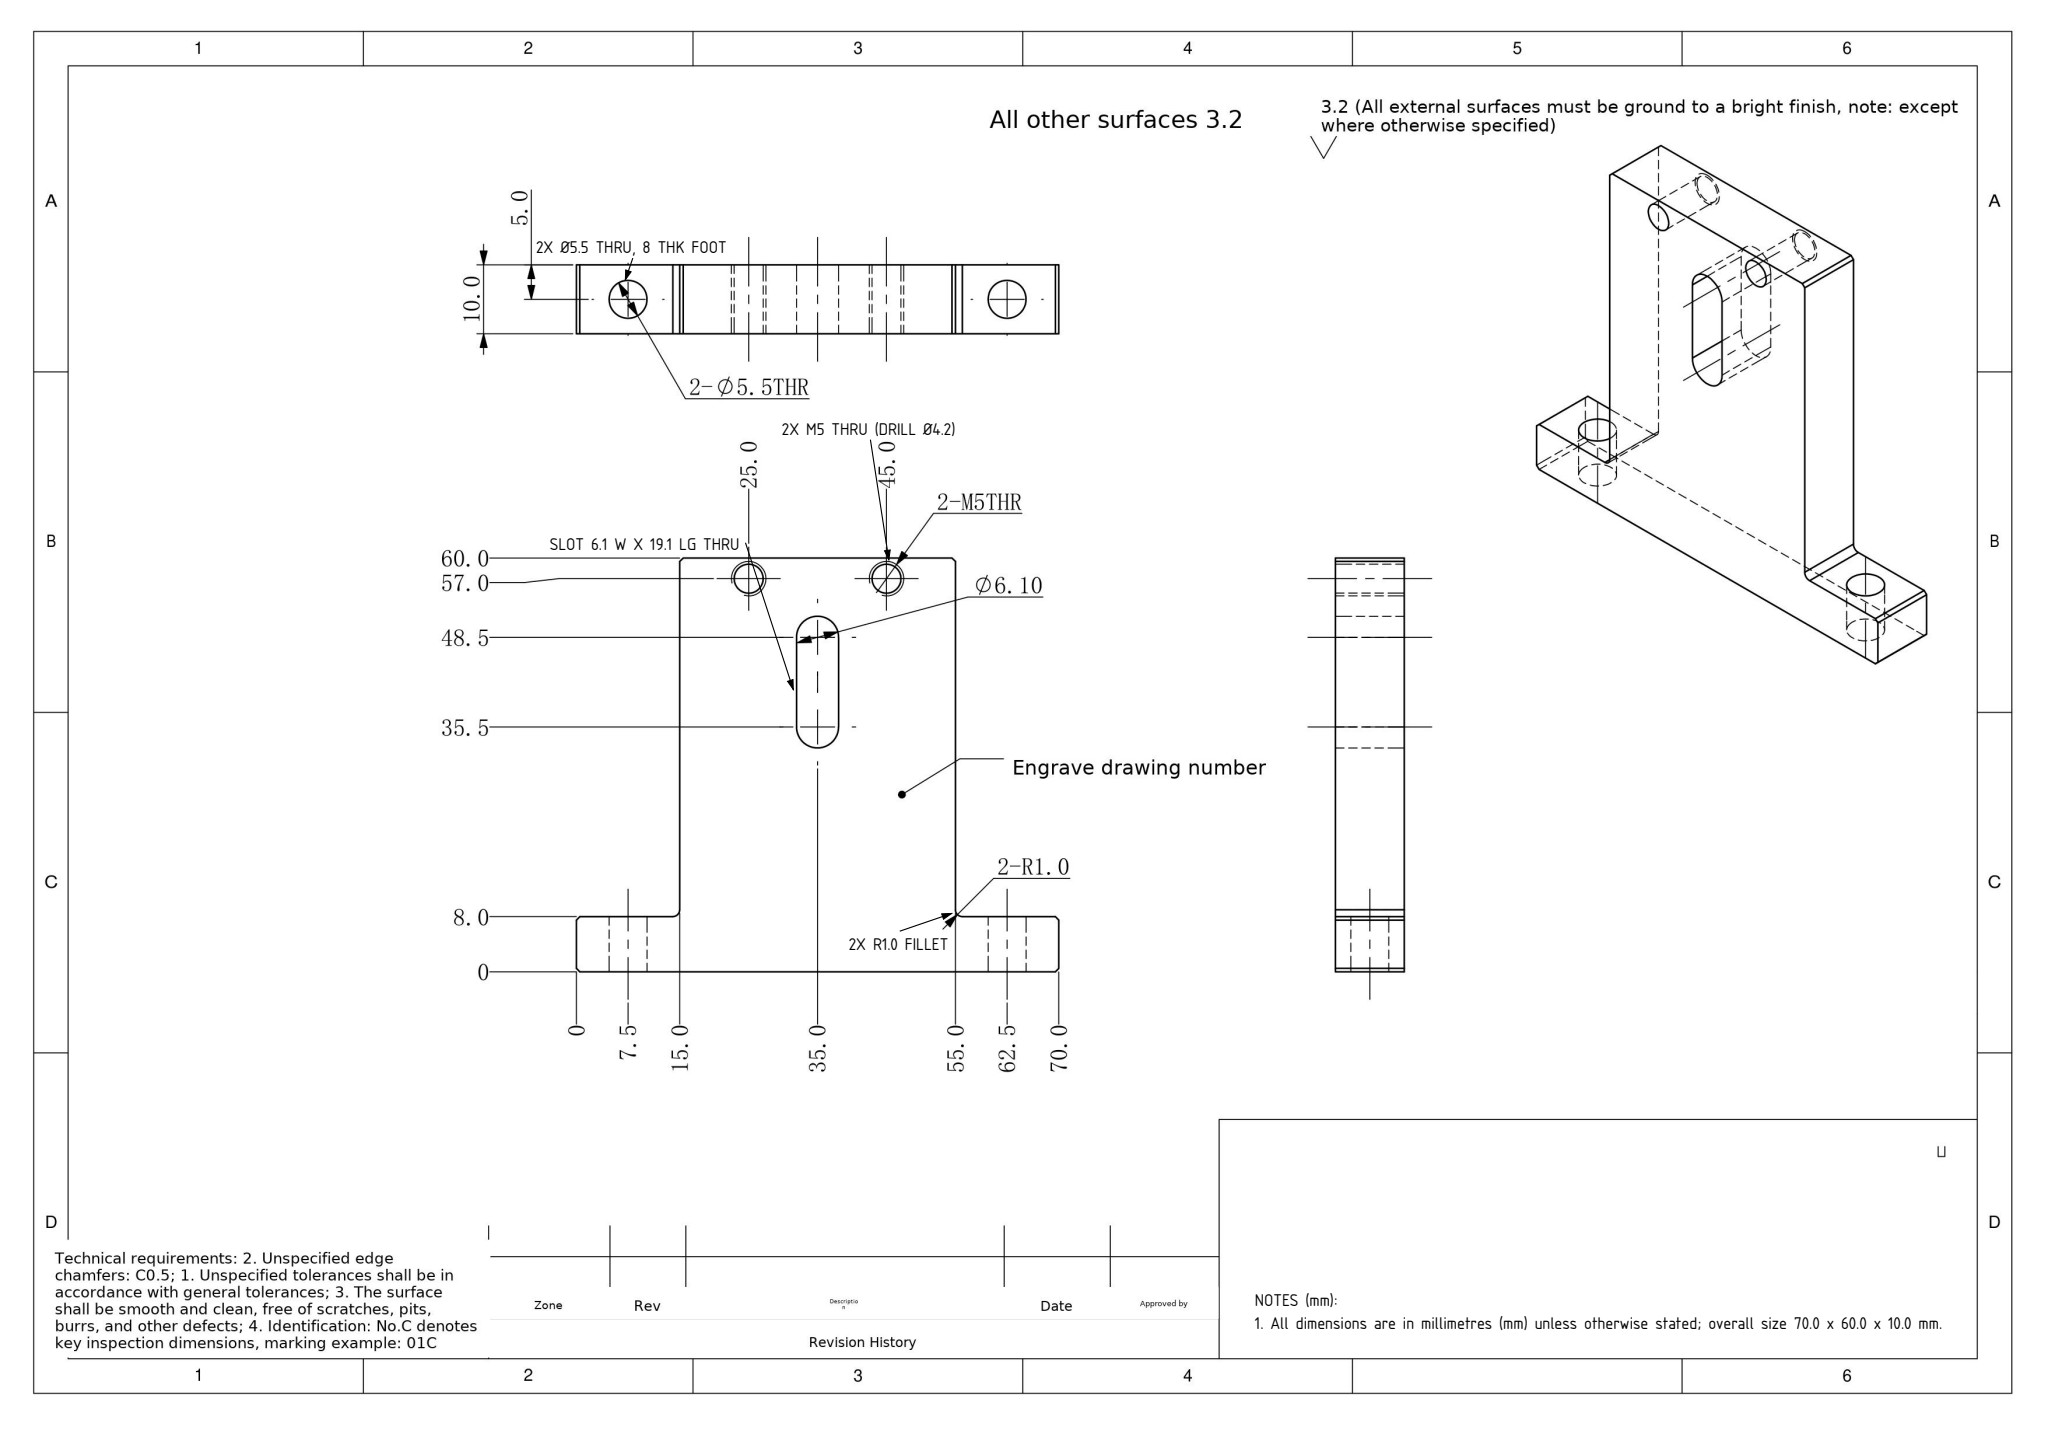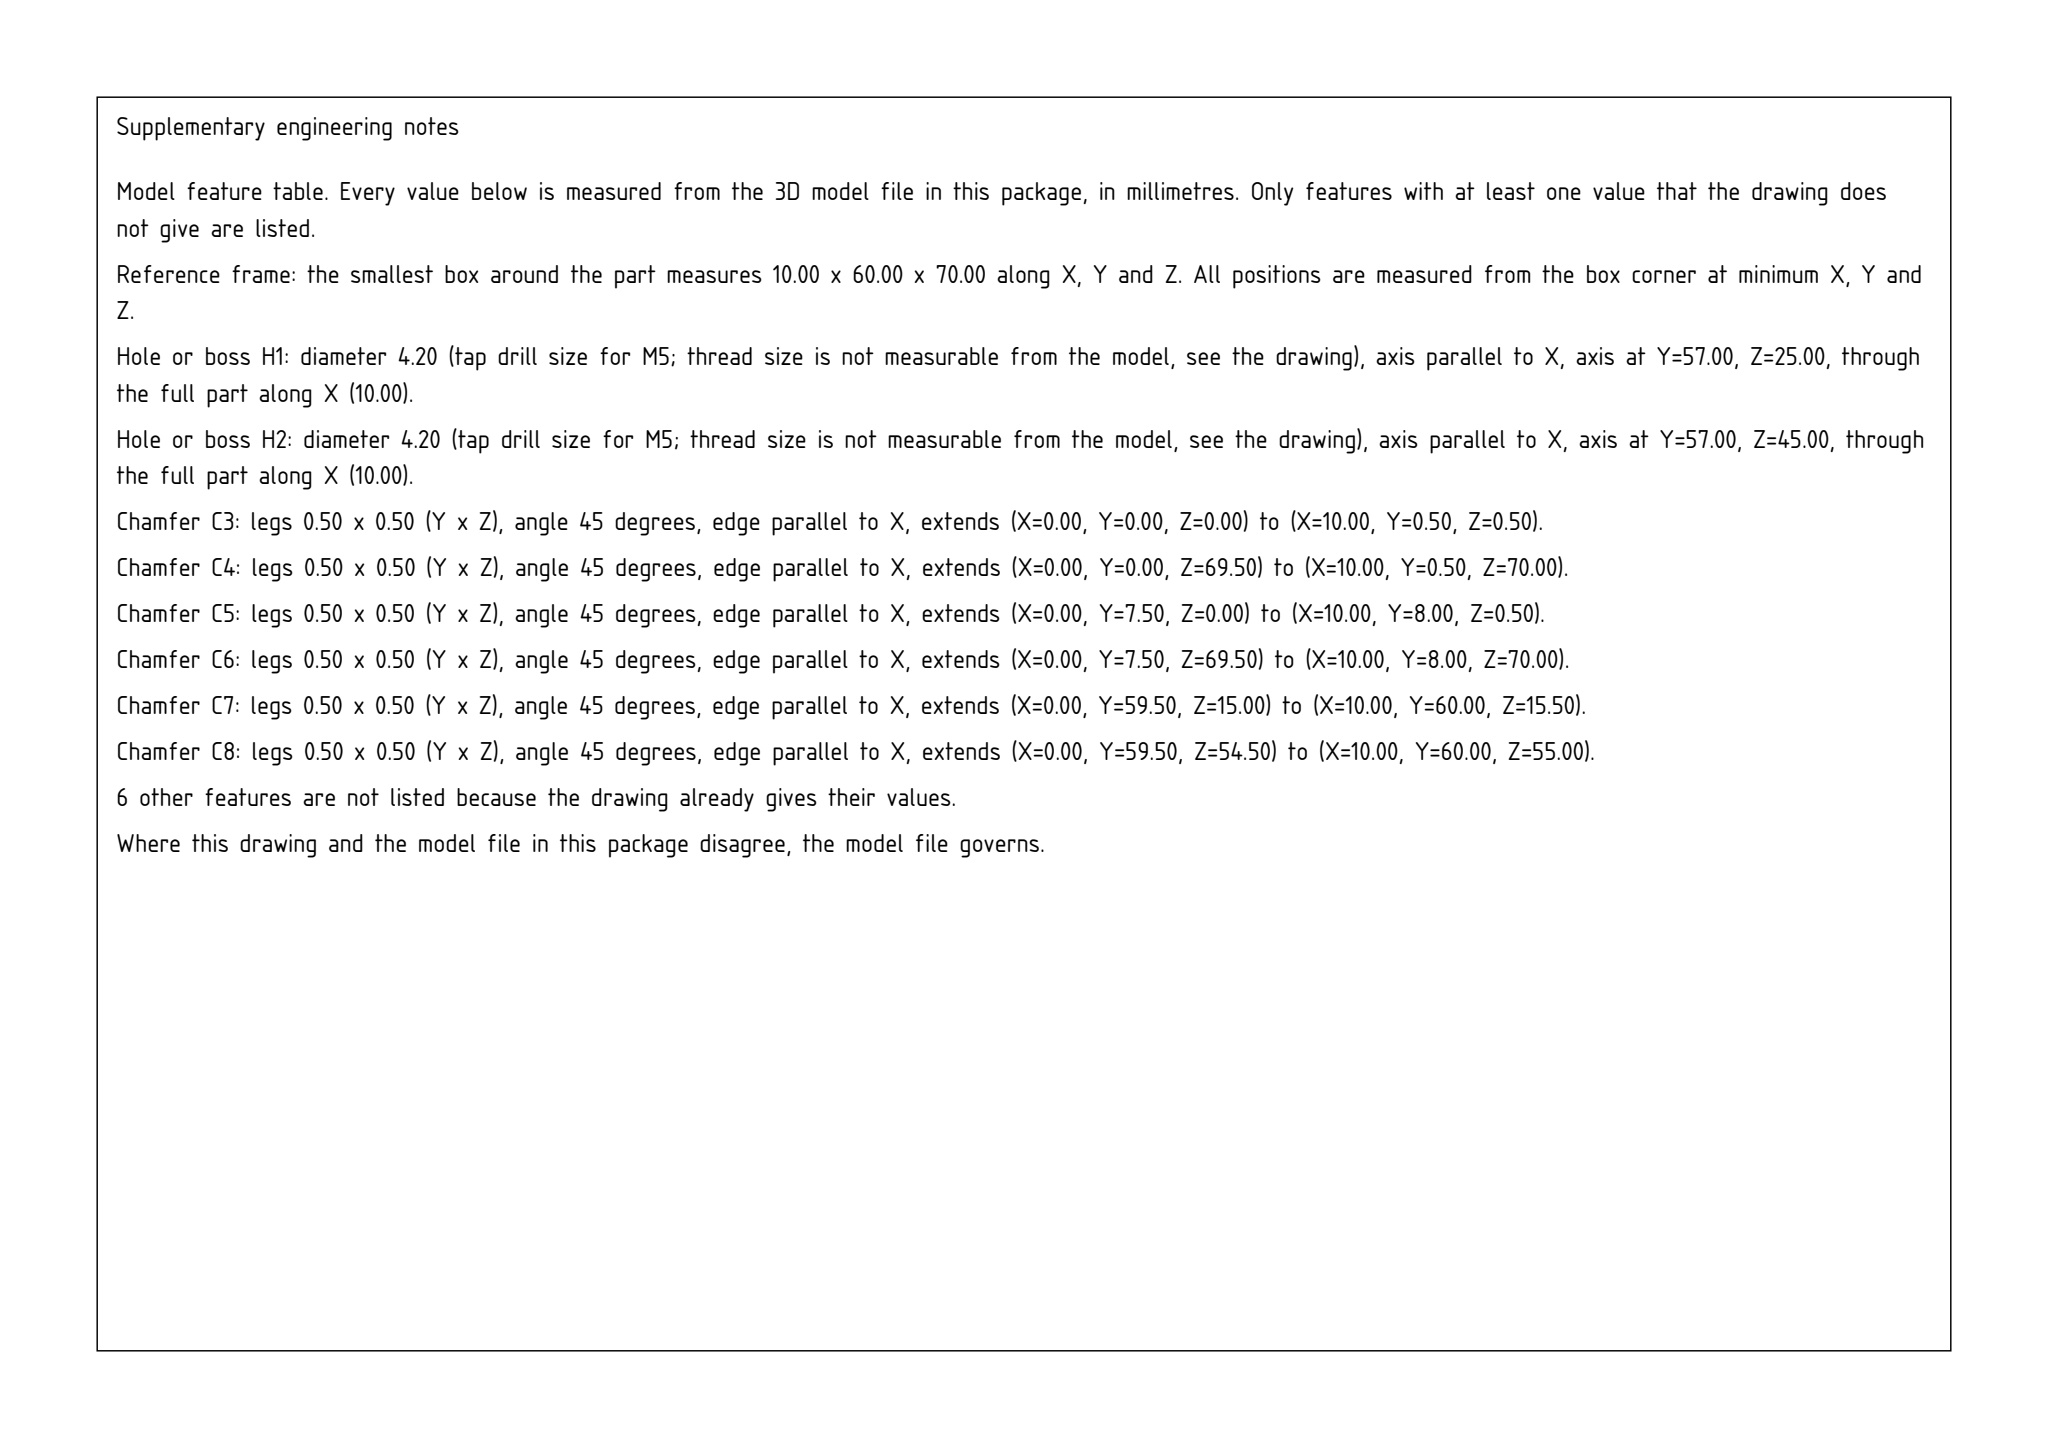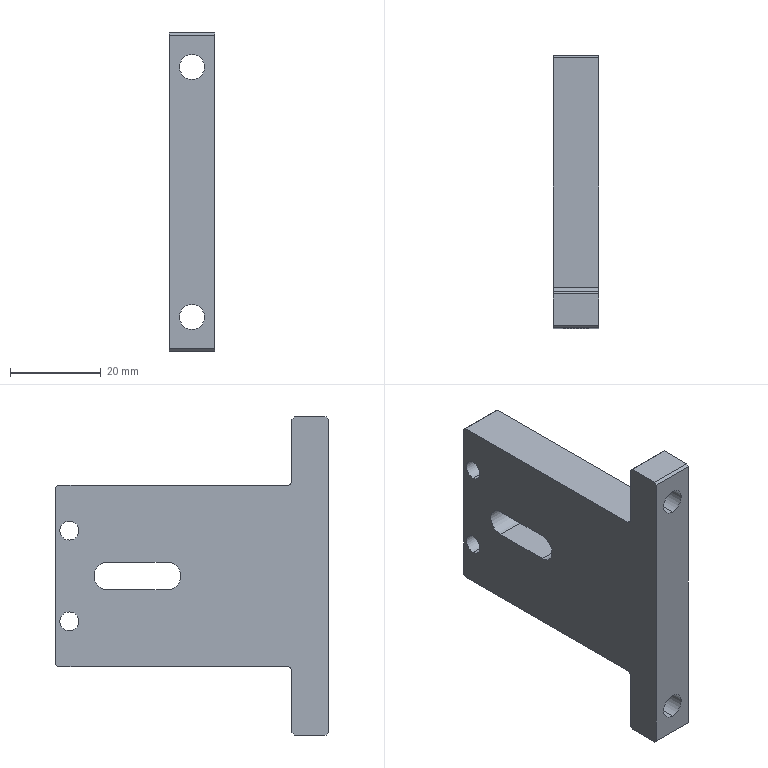Part | SolidWorks | mm | 1 solid | 30 faces | box 10 x 60 x 70 mm | volume 24654 mm3 | plane 18 | cylinder 12 | commonest cylinder face diameters 4.2 x4 5.5 x4 6.1 x2 2 x2
Drawing notes:
All dimensions are in millimetres (mm) unless otherwise stated; overall size 70.0 x 60.0 x 10.0 mm. | from the solid: STEP model units mm, bbox_xyz [10.0, 60.0, 70.0]
2X Ø5.5 THRU 8 THK FEET, AT 7.5 & 62.5 FROM LH END | from the solid: hole/bore dia 5.5, axis y, at x=5.0, z=7.5 and z=62.5, from y=0.0 to 8.0 (full 8 thk foot)
2X M5 THRU 10 THK PLATE (TAP DRILL Ø4.2) | from the solid: hole/bore dia 4.2, axis x, at y=57.0, z=25.0 and 45.0, from x=0.0 to 10.0 = full 10 plate thk
SLOT 6.1 WIDE x 19.1 LG THRU, R3.05 ENDS, CTRS 13 APART | from the solid: two 180 deg arcs dia 6.1, axis x, at z=35.0, y=35.5 and 48.5, from x=0.0 to 10.0; flats z=32.0 & 38.1
2-R1.0 = FILLETS AT FOOT/PLATE JOINT, NO Ø2.0 HOLES | from the solid: concave 90 deg arcs dia 2.0 (R1.0), axis x, at y=9.0, z=14.0 and 56.0, full 10 width; only holes are Ø5.5 and Ø4.2
build123d program:
from build123d import *

# Parameters (mm, degrees)
SKETCH1_W                      = 40
SKETCH1_H                      = 60
BOSS_EXTRUDE1_DEPTH            = 10
SKETCH2_W                      = 15
SKETCH2_H                      = 8
BOSS_EXTRUDE2_DEPTH            = 10
F_5_5_5_5_DIAMETER_HOLE1_D     = 5.5
F_5_5_5_5_DIAMETER_HOLE1_DEPTH = 30
F_5_5_5_5_DIAMETER_HOLE1_TIP   = 1.652
FILLET1_R                      = 1
CHAMFER1_SIZE                  = 0.5
M5_TAPPED_HOLE1_D              = 4.2
M5_TAPPED_HOLE1_DEPTH          = 12.4
M5_TAPPED_HOLE1_TIP            = 1.262


with BuildPart() as part:
    # Sketch1 → Boss-Extrude1 (new body)
    with BuildSketch(Plane(origin=(0, 0, 0), x_dir=(0, 0, -1), z_dir=(1, 0, 0))):
        Rectangle(SKETCH1_W, SKETCH1_H)
        with BuildLine():
            Line((3.05, 18.5), (3.05, 5.5))
            ThreePointArc((3.05, 5.5), (0, 2.45), (-3.05, 5.5))
            Line((-3.05, 5.5), (-3.05, 18.5))
            ThreePointArc((-3.05, 18.5), (0, 21.55), (3.05, 18.5))
        make_face(mode=Mode.SUBTRACT)
    extrude(amount=BOSS_EXTRUDE1_DEPTH)

    # Sketch2 → Boss-Extrude2 (add)
    with BuildSketch(Plane(origin=(10, 0, 0), x_dir=(0, 0, -1), z_dir=(1, 0, 0))):
        with Locations((-27.5, -26)):
            Rectangle(SKETCH2_W, SKETCH2_H)
        with Locations((27.5, -26)):
            Rectangle(SKETCH2_W, SKETCH2_H)
    extrude(amount=-BOSS_EXTRUDE2_DEPTH)

    # 5.5 _5.5_ Diameter Hole1
    with Locations(Plane(origin=(5, -22, 27.5), x_dir=(0, 0, 1), z_dir=(0, 1, 0))):
        with Locations((0, 0), (-55, 0)):
            Hole(F_5_5_5_5_DIAMETER_HOLE1_D / 2, depth=F_5_5_5_5_DIAMETER_HOLE1_DEPTH)
            with Locations((0, 0, -(F_5_5_5_5_DIAMETER_HOLE1_DEPTH + F_5_5_5_5_DIAMETER_HOLE1_TIP / 2))):  # 118° drill point
                Cone(0, F_5_5_5_5_DIAMETER_HOLE1_D / 2, F_5_5_5_5_DIAMETER_HOLE1_TIP, mode=Mode.SUBTRACT)

    # Fillet1
    fillet1_edges = [part.edges().sort_by_distance(p)[0] for p in [
        (5, -22, -20),
        (5, -22, 20),
    ]]
    fillet(fillet1_edges, radius=FILLET1_R)

    # Chamfer1
    chamfer1_edges = [part.edges().sort_by_distance(p)[0] for p in [
        (5, -30, -35),
        (5, -30, 35),
        (5, -22, -35),
        (5, -22, 35),
        (5, 30, -20),
        (5, 30, 20),
    ]]
    chamfer(chamfer1_edges, length=CHAMFER1_SIZE)

    # M5 Tapped Hole1
    with Locations(Plane.ZY):
        with Locations((-10, 27), (10, 27)):
            Hole(M5_TAPPED_HOLE1_D / 2, depth=M5_TAPPED_HOLE1_DEPTH)
            with Locations((0, 0, -(M5_TAPPED_HOLE1_DEPTH + M5_TAPPED_HOLE1_TIP / 2))):  # 118° drill point
                Cone(0, M5_TAPPED_HOLE1_D / 2, M5_TAPPED_HOLE1_TIP, mode=Mode.SUBTRACT)


solid = part.part